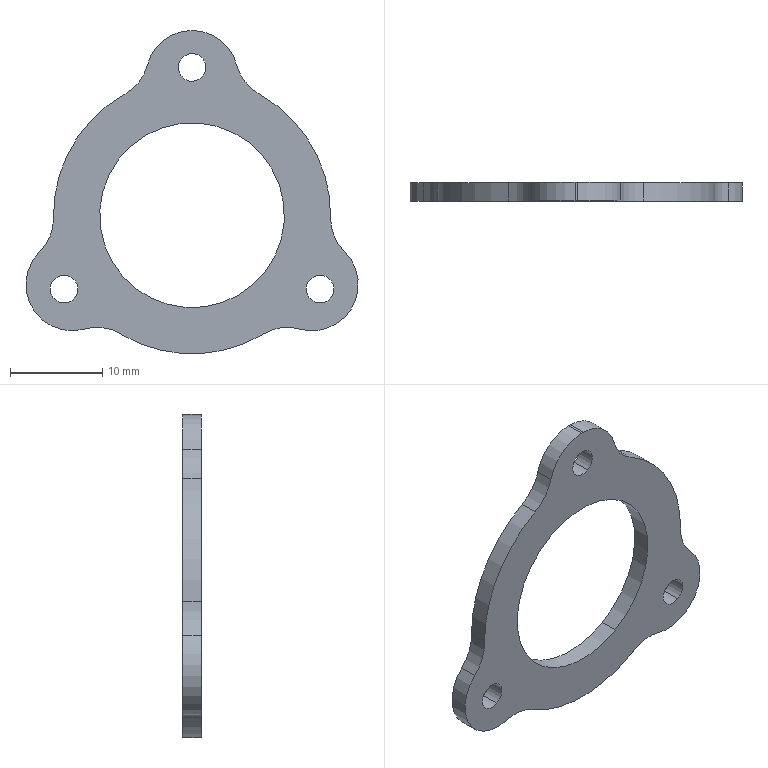Component | SolidWorks | NozzleGasket1-1 | 1 solid | 27 faces | box 35.98 x 2 x 35 mm | volume 1008 mm3 | cylinder 25 | plane 2 | commonest cylinder face diameters 10 x12 3 x6 30 x4 20 x2 40 x1
build123d program:
from build123d import *

# Parameters (mm, degrees)
SKETCH1_R           = 10
BOSS_EXTRUDE1_DEPTH = 2
FILLET1_R           = 5
CUT_EXTRUDE1_REACH  = 28.976
SKETCH2_R           = 1.5


with BuildPart() as part:
    # Sketch1 → Boss-Extrude1 (new body)
    with BuildSketch(Plane.XY):
        with BuildLine():
            ThreePointArc((4.93, 14.167), (0, 20), (-4.93, 14.167))
            ThreePointArc((-4.93, 14.167), (-12.991, 7.499), (-14.733, -2.815))
            ThreePointArc((-14.733, -2.815), (-17.319, -10.001), (-9.802, -11.354))
            ThreePointArc((-9.802, -11.354), (0.001646, -15), (9.805, -11.352))
            ThreePointArc((9.805, -11.352), (17.322, -9.999), (14.734, -2.812))
            ThreePointArc((14.734, -2.812), (12.99, 7.501), (4.93, 14.167))
        make_face()
        Circle(SKETCH1_R, mode=Mode.SUBTRACT)
    extrude(amount=BOSS_EXTRUDE1_DEPTH)

    # Fillet1
    fillet1_edges = [part.edges().sort_by_distance(p)[0] for p in [
        (14.734, -2.812, 1),
        (9.805, -11.352, 1),
        (-9.802, -11.354, 1),
        (-14.733, -2.815, 1),
        (-4.93, 14.167, 1),
        (4.93, 14.167, 1),
    ]]
    fillet(fillet1_edges, radius=FILLET1_R)

    # Sketch2 → Cut-Extrude1 (cut, up to next)
    with BuildSketch(Plane.XY.offset(2), mode=Mode.PRIVATE) as cut_extrude1_sk1:
        with Locations((0, 16)):
            Circle(SKETCH2_R)
    cut_extrude1_tool1 = extrude(cut_extrude1_sk1.sketch, amount=-CUT_EXTRUDE1_REACH, mode=Mode.PRIVATE) & part.part
    # Sketch2 → Cut-Extrude1 (cut, up to next)
    with BuildSketch(Plane.XY.offset(2), mode=Mode.PRIVATE) as cut_extrude1_sk2:
        with Locations((13.856, -8)):
            Circle(SKETCH2_R)
    cut_extrude1_tool2 = extrude(cut_extrude1_sk2.sketch, amount=-CUT_EXTRUDE1_REACH, mode=Mode.PRIVATE) & part.part
    # Sketch2 → Cut-Extrude1 (cut, up to next)
    with BuildSketch(Plane.XY.offset(2), mode=Mode.PRIVATE) as cut_extrude1_sk3:
        with Locations((-13.856, -8)):
            Circle(SKETCH2_R)
    cut_extrude1_tool3 = extrude(cut_extrude1_sk3.sketch, amount=-CUT_EXTRUDE1_REACH, mode=Mode.PRIVATE) & part.part
    add(cut_extrude1_tool1.solids().sort_by_distance((0, 16, 2))[0], mode=Mode.SUBTRACT)
    add(cut_extrude1_tool2.solids().sort_by_distance((13.856, -8, 2))[0], mode=Mode.SUBTRACT)
    add(cut_extrude1_tool3.solids().sort_by_distance((-13.856, -8, 2))[0], mode=Mode.SUBTRACT)


solid = part.part

# Placed as in the assembly
solid = solid.moved(Location((-5.982, -9.494, 160.001), (90, 0, 0)))
STEP:
#1=COLOUR_RGB('',0.7922,0.8196,0.9333);
#2=FILL_AREA_STYLE_COLOUR('',#1);
#3=FILL_AREA_STYLE('',(#2));
#4=SURFACE_STYLE_FILL_AREA(#3);
#5=SURFACE_SIDE_STYLE('',(#4));
#6=SURFACE_STYLE_USAGE(.BOTH.,#5);
#7=PRESENTATION_STYLE_ASSIGNMENT((#6));
#8=CARTESIAN_POINT('',(-0.8105,-0.3738,6.035));
#9=VERTEX_POINT('',#8);
#10=CARTESIAN_POINT('',(-0.7515,-0.3738,5.933));
#11=VERTEX_POINT('',#10);
#12=CARTESIAN_POINT('',(-0.781,-0.3738,5.984));
#13=DIRECTION('',(0.,1.,0.));
#14=DIRECTION('',(-0.5,0.,0.866));
#15=AXIS2_PLACEMENT_3D('',#12,#13,#14);
#16=CIRCLE('',#15,0.05906);
#17=EDGE_CURVE('',#9,#11,#16,.T.);
#18=ORIENTED_EDGE('',*,*,#17,.T.);
#19=CARTESIAN_POINT('',(-0.7515,-0.4525,5.933));
#20=VERTEX_POINT('',#19);
#21=CARTESIAN_POINT('',(-0.7515,-0.3737,5.933));
#22=DIRECTION('',(-0.,-1.,-0.));
#23=VECTOR('',#22,39.37);
#24=LINE('',#21,#23);
#25=EDGE_CURVE('',#11,#20,#24,.T.);
#26=ORIENTED_EDGE('',*,*,#25,.T.);
#27=CARTESIAN_POINT('',(-0.8105,-0.4525,6.035));
#28=VERTEX_POINT('',#27);
#29=CARTESIAN_POINT('',(-0.781,-0.4525,5.984));
#30=DIRECTION('',(-0.,-1.,-0.));
#31=DIRECTION('',(-0.5,0.,0.866));
#32=AXIS2_PLACEMENT_3D('',#29,#30,#31);
#33=CIRCLE('',#32,0.05906);
#34=EDGE_CURVE('',#20,#28,#33,.T.);
#35=ORIENTED_EDGE('',*,*,#34,.T.);
#36=CARTESIAN_POINT('',(-0.8105,-0.3737,6.035));
#37=DIRECTION('',(-0.,-1.,-0.));
#38=VECTOR('',#37,39.37);
#39=LINE('',#36,#38);
#40=EDGE_CURVE('',#9,#28,#39,.T.);
#41=ORIENTED_EDGE('',*,*,#40,.F.);
#42=EDGE_LOOP('',(#18,#26,#35,#41));
#43=FACE_OUTER_BOUND('',#42,.T.);
#44=CARTESIAN_POINT('',(-0.781,-0.3737,5.984));
#45=DIRECTION('',(-0.,-1.,-0.));
#46=DIRECTION('',(-0.5,0.,0.866));
#47=AXIS2_PLACEMENT_3D('',#44,#45,#46);
#48=CYLINDRICAL_SURFACE('',#47,0.05906);
#49=ADVANCED_FACE('',(#43),#48,.F.);
#50=CARTESIAN_POINT('',(-0.265,-0.3738,6.98));
#51=VERTEX_POINT('',#50);
#52=CARTESIAN_POINT('',(-0.2059,-0.3738,6.878));
#53=VERTEX_POINT('',#52);
#54=CARTESIAN_POINT('',(-0.2355,-0.3738,6.929));
#55=DIRECTION('',(0.,1.,0.));
#56=DIRECTION('',(-0.5,0.,0.866));
#57=AXIS2_PLACEMENT_3D('',#54,#55,#56);
#58=CIRCLE('',#57,0.05906);
#59=EDGE_CURVE('',#51,#53,#58,.T.);
#60=ORIENTED_EDGE('',*,*,#59,.T.);
#61=CARTESIAN_POINT('',(-0.2059,-0.4525,6.878));
#62=VERTEX_POINT('',#61);
#63=CARTESIAN_POINT('',(-0.2059,-0.3737,6.878));
#64=DIRECTION('',(-0.,-1.,-0.));
#65=VECTOR('',#64,39.37);
#66=LINE('',#63,#65);
#67=EDGE_CURVE('',#53,#62,#66,.T.);
#68=ORIENTED_EDGE('',*,*,#67,.T.);
#69=CARTESIAN_POINT('',(-0.265,-0.4525,6.98));
#70=VERTEX_POINT('',#69);
#71=CARTESIAN_POINT('',(-0.2355,-0.4525,6.929));
#72=DIRECTION('',(-0.,-1.,-0.));
#73=DIRECTION('',(-0.5,0.,0.866));
#74=AXIS2_PLACEMENT_3D('',#71,#72,#73);
#75=CIRCLE('',#74,0.05906);
#76=EDGE_CURVE('',#62,#70,#75,.T.);
#77=ORIENTED_EDGE('',*,*,#76,.T.);
#78=CARTESIAN_POINT('',(-0.265,-0.3737,6.98));
#79=DIRECTION('',(-0.,-1.,-0.));
#80=VECTOR('',#79,39.37);
#81=LINE('',#78,#80);
#82=EDGE_CURVE('',#51,#70,#81,.T.);
#83=ORIENTED_EDGE('',*,*,#82,.F.);
#84=EDGE_LOOP('',(#60,#68,#77,#83));
#85=FACE_OUTER_BOUND('',#84,.T.);
#86=CARTESIAN_POINT('',(-0.2355,-0.3737,6.929));
#87=DIRECTION('',(-0.,-1.,-0.));
#88=DIRECTION('',(-0.5,0.,0.866));
#89=AXIS2_PLACEMENT_3D('',#86,#87,#88);
#90=CYLINDRICAL_SURFACE('',#89,0.05906);
#91=ADVANCED_FACE('',(#85),#90,.F.);
#92=CARTESIAN_POINT('',(0.2805,-0.3738,6.035));
#93=VERTEX_POINT('',#92);
#94=CARTESIAN_POINT('',(0.3396,-0.3738,5.933));
#95=VERTEX_POINT('',#94);
#96=CARTESIAN_POINT('',(0.3101,-0.3738,5.984));
#97=DIRECTION('',(0.,1.,0.));
#98=DIRECTION('',(-0.5,0.,0.866));
#99=AXIS2_PLACEMENT_3D('',#96,#97,#98);
#100=CIRCLE('',#99,0.05906);
#101=EDGE_CURVE('',#93,#95,#100,.T.);
#102=ORIENTED_EDGE('',*,*,#101,.T.);
#103=CARTESIAN_POINT('',(0.3396,-0.4525,5.933));
#104=VERTEX_POINT('',#103);
#105=CARTESIAN_POINT('',(0.3396,-0.3737,5.933));
#106=DIRECTION('',(-0.,-1.,-0.));
#107=VECTOR('',#106,39.37);
#108=LINE('',#105,#107);
#109=EDGE_CURVE('',#95,#104,#108,.T.);
#110=ORIENTED_EDGE('',*,*,#109,.T.);
#111=CARTESIAN_POINT('',(0.2805,-0.4525,6.035));
#112=VERTEX_POINT('',#111);
#113=CARTESIAN_POINT('',(0.3101,-0.4525,5.984));
#114=DIRECTION('',(-0.,-1.,-0.));
#115=DIRECTION('',(-0.5,0.,0.866));
#116=AXIS2_PLACEMENT_3D('',#113,#114,#115);
#117=CIRCLE('',#116,0.05906);
#118=EDGE_CURVE('',#104,#112,#117,.T.);
#119=ORIENTED_EDGE('',*,*,#118,.T.);
#120=CARTESIAN_POINT('',(0.2805,-0.3737,6.035));
#121=DIRECTION('',(-0.,-1.,-0.));
#122=VECTOR('',#121,39.37);
#123=LINE('',#120,#122);
#124=EDGE_CURVE('',#93,#112,#123,.T.);
#125=ORIENTED_EDGE('',*,*,#124,.F.);
#126=EDGE_LOOP('',(#102,#110,#119,#125));
#127=FACE_OUTER_BOUND('',#126,.T.);
#128=CARTESIAN_POINT('',(0.3101,-0.3737,5.984));
#129=DIRECTION('',(-0.,-1.,-0.));
#130=DIRECTION('',(-0.5,0.,0.866));
#131=AXIS2_PLACEMENT_3D('',#128,#129,#130);
#132=CYLINDRICAL_SURFACE('',#131,0.05906);
#133=ADVANCED_FACE('',(#127),#132,.F.);
#134=CARTESIAN_POINT('',(0.07226,-0.3738,5.795));
#135=VERTEX_POINT('',#134);
#136=CARTESIAN_POINT('',(0.06914,-0.3738,5.793));
#137=VERTEX_POINT('',#136);
#138=CARTESIAN_POINT('',(0.1707,-0.3738,5.625));
#139=DIRECTION('',(-0.,-1.,-0.));
#140=DIRECTION('',(-0.5,-0.,0.866));
#141=AXIS2_PLACEMENT_3D('',#138,#139,#140);
#142=CIRCLE('',#141,0.1969);
#143=EDGE_CURVE('',#135,#137,#142,.T.);
#144=ORIENTED_EDGE('',*,*,#143,.F.);
#145=CARTESIAN_POINT('',(0.07226,-0.4525,5.795));
#146=VERTEX_POINT('',#145);
#147=CARTESIAN_POINT('',(0.07226,-0.4525,5.795));
#148=DIRECTION('',(-0.,-1.,-0.));
#149=VECTOR('',#148,39.37);
#150=LINE('',#147,#149);
#151=EDGE_CURVE('',#135,#146,#150,.T.);
#152=ORIENTED_EDGE('',*,*,#151,.T.);
#153=CARTESIAN_POINT('',(0.06914,-0.4525,5.793));
#154=VERTEX_POINT('',#153);
#155=CARTESIAN_POINT('',(0.1707,-0.4525,5.625));
#156=DIRECTION('',(0.,1.,0.));
#157=DIRECTION('',(-0.5,-0.,0.866));
#158=AXIS2_PLACEMENT_3D('',#155,#156,#157);
#159=CIRCLE('',#158,0.1969);
#160=EDGE_CURVE('',#154,#146,#159,.T.);
#161=ORIENTED_EDGE('',*,*,#160,.F.);
#162=CARTESIAN_POINT('',(0.06914,-0.4525,5.793));
#163=DIRECTION('',(-0.,-1.,-0.));
#164=VECTOR('',#163,39.37);
#165=LINE('',#162,#164);
#166=EDGE_CURVE('',#137,#154,#165,.T.);
#167=ORIENTED_EDGE('',*,*,#166,.F.);
#168=EDGE_LOOP('',(#144,#152,#161,#167));
#169=FACE_OUTER_BOUND('',#168,.T.);
#170=CARTESIAN_POINT('',(0.1707,-0.4525,5.625));
#171=DIRECTION('',(-0.,-1.,-0.));
#172=DIRECTION('',(-0.5,-0.,0.866));
#173=AXIS2_PLACEMENT_3D('',#170,#171,#172);
#174=CYLINDRICAL_SURFACE('',#173,0.1969);
#175=ADVANCED_FACE('',(#169),#174,.F.);
#176=CARTESIAN_POINT('',(-0.03862,-0.4525,5.958));
#177=VERTEX_POINT('',#176);
#178=CARTESIAN_POINT('',(-0.4323,-0.4525,6.64));
#179=VERTEX_POINT('',#178);
#180=CARTESIAN_POINT('',(-0.2355,-0.4525,6.299));
#181=DIRECTION('',(-0.,-1.,-0.));
#182=DIRECTION('',(-0.5,-0.,0.866));
#183=AXIS2_PLACEMENT_3D('',#180,#181,#182);
#184=CIRCLE('',#183,0.3937);
#185=EDGE_CURVE('',#177,#179,#184,.T.);
#186=ORIENTED_EDGE('',*,*,#185,.T.);
#187=CARTESIAN_POINT('',(-0.4323,-0.3738,6.64));
#188=VERTEX_POINT('',#187);
#189=CARTESIAN_POINT('',(-0.4323,-0.4525,6.64));
#190=DIRECTION('',(0.,1.,0.));
#191=VECTOR('',#190,39.37);
#192=LINE('',#189,#191);
#193=EDGE_CURVE('',#179,#188,#192,.T.);
#194=ORIENTED_EDGE('',*,*,#193,.T.);
#195=CARTESIAN_POINT('',(-0.03862,-0.3738,5.958));
#196=VERTEX_POINT('',#195);
#197=CARTESIAN_POINT('',(-0.2355,-0.3738,6.299));
#198=DIRECTION('',(-0.,-1.,-0.));
#199=DIRECTION('',(-0.5,-0.,0.866));
#200=AXIS2_PLACEMENT_3D('',#197,#198,#199);
#201=CIRCLE('',#200,0.3937);
#202=EDGE_CURVE('',#196,#188,#201,.T.);
#203=ORIENTED_EDGE('',*,*,#202,.F.);
#204=CARTESIAN_POINT('',(-0.03862,-0.4525,5.958));
#205=DIRECTION('',(0.,1.,0.));
#206=VECTOR('',#205,39.37);
#207=LINE('',#204,#206);
#208=EDGE_CURVE('',#177,#196,#207,.T.);
#209=ORIENTED_EDGE('',*,*,#208,.F.);
#210=EDGE_LOOP('',(#186,#194,#203,#209));
#211=FACE_OUTER_BOUND('',#210,.T.);
#212=CARTESIAN_POINT('',(-0.2355,-0.4525,6.299));
#213=DIRECTION('',(0.,1.,0.));
#214=DIRECTION('',(0.5,0.,-0.866));
#215=AXIS2_PLACEMENT_3D('',#212,#213,#214);
#216=CYLINDRICAL_SURFACE('',#215,0.3937);
#217=ADVANCED_FACE('',(#211),#216,.F.);
#218=CARTESIAN_POINT('',(0.3744,-0.4525,5.834));
#219=VERTEX_POINT('',#218);
#220=CARTESIAN_POINT('',(0.4139,-0.4525,6.144));
#221=VERTEX_POINT('',#220);
#222=CARTESIAN_POINT('',(0.276,-0.4525,6.004));
#223=DIRECTION('',(-0.,-1.,-0.));
#224=DIRECTION('',(-0.5,-0.,0.866));
#225=AXIS2_PLACEMENT_3D('',#222,#223,#224);
#226=CIRCLE('',#225,0.1969);
#227=EDGE_CURVE('',#219,#221,#226,.T.);
#228=ORIENTED_EDGE('',*,*,#227,.F.);
#229=CARTESIAN_POINT('',(0.3744,-0.3738,5.834));
#230=VERTEX_POINT('',#229);
#231=CARTESIAN_POINT('',(0.3744,-0.4525,5.834));
#232=DIRECTION('',(0.,1.,0.));
#233=VECTOR('',#232,39.37);
#234=LINE('',#231,#233);
#235=EDGE_CURVE('',#219,#230,#234,.T.);
#236=ORIENTED_EDGE('',*,*,#235,.T.);
#237=CARTESIAN_POINT('',(0.4139,-0.3738,6.144));
#238=VERTEX_POINT('',#237);
#239=CARTESIAN_POINT('',(0.276,-0.3738,6.004));
#240=DIRECTION('',(-0.,-1.,-0.));
#241=DIRECTION('',(-0.5,-0.,0.866));
#242=AXIS2_PLACEMENT_3D('',#239,#240,#241);
#243=CIRCLE('',#242,0.1969);
#244=EDGE_CURVE('',#230,#238,#243,.T.);
#245=ORIENTED_EDGE('',*,*,#244,.T.);
#246=CARTESIAN_POINT('',(0.4139,-0.4525,6.144));
#247=DIRECTION('',(-0.,-1.,-0.));
#248=VECTOR('',#247,39.37);
#249=LINE('',#246,#248);
#250=EDGE_CURVE('',#238,#221,#249,.T.);
#251=ORIENTED_EDGE('',*,*,#250,.T.);
#252=EDGE_LOOP('',(#228,#236,#245,#251));
#253=FACE_OUTER_BOUND('',#252,.T.);
#254=CARTESIAN_POINT('',(0.276,-0.4525,6.004));
#255=DIRECTION('',(0.,1.,0.));
#256=DIRECTION('',(0.5,0.,-0.866));
#257=AXIS2_PLACEMENT_3D('',#254,#255,#256);
#258=CYLINDRICAL_SURFACE('',#257,0.1969);
#259=ADVANCED_FACE('',(#253),#258,.T.);
#260=CARTESIAN_POINT('',(0.05981,-0.4525,5.788));
#261=VERTEX_POINT('',#260);
#262=CARTESIAN_POINT('',(-0.2355,-0.4525,6.299));
#263=DIRECTION('',(-0.,-1.,-0.));
#264=DIRECTION('',(-0.5,-0.,0.866));
#265=AXIS2_PLACEMENT_3D('',#262,#263,#264);
#266=CIRCLE('',#265,0.5906);
#267=EDGE_CURVE('',#261,#154,#266,.T.);
#268=ORIENTED_EDGE('',*,*,#267,.F.);
#269=CARTESIAN_POINT('',(0.05981,-0.3738,5.788));
#270=VERTEX_POINT('',#269);
#271=CARTESIAN_POINT('',(0.05981,-0.4525,5.788));
#272=DIRECTION('',(0.,1.,0.));
#273=VECTOR('',#272,39.37);
#274=LINE('',#271,#273);
#275=EDGE_CURVE('',#261,#270,#274,.T.);
#276=ORIENTED_EDGE('',*,*,#275,.T.);
#277=CARTESIAN_POINT('',(-0.2355,-0.3738,6.299));
#278=DIRECTION('',(-0.,-1.,-0.));
#279=DIRECTION('',(-0.5,-0.,0.866));
#280=AXIS2_PLACEMENT_3D('',#277,#278,#279);
#281=CIRCLE('',#280,0.5906);
#282=EDGE_CURVE('',#270,#137,#281,.T.);
#283=ORIENTED_EDGE('',*,*,#282,.T.);
#284=ORIENTED_EDGE('',*,*,#166,.T.);
#285=EDGE_LOOP('',(#268,#276,#283,#284));
#286=FACE_OUTER_BOUND('',#285,.T.);
#287=CARTESIAN_POINT('',(-0.2355,-0.4525,6.299));
#288=DIRECTION('',(0.,1.,0.));
#289=DIRECTION('',(0.5,0.,-0.866));
#290=AXIS2_PLACEMENT_3D('',#287,#288,#289);
#291=CYLINDRICAL_SURFACE('',#290,0.5906);
#292=ADVANCED_FACE('',(#286),#291,.T.);
#293=CARTESIAN_POINT('',(-0.5214,-0.4525,6.816));
#294=VERTEX_POINT('',#293);
#295=CARTESIAN_POINT('',(-0.8259,-0.4525,6.288));
#296=VERTEX_POINT('',#295);
#297=CARTESIAN_POINT('',(-0.2355,-0.4525,6.299));
#298=DIRECTION('',(-0.,-1.,-0.));
#299=DIRECTION('',(-0.5,-0.,0.866));
#300=AXIS2_PLACEMENT_3D('',#297,#298,#299);
#301=CIRCLE('',#300,0.5906);
#302=EDGE_CURVE('',#294,#296,#301,.T.);
#303=ORIENTED_EDGE('',*,*,#302,.F.);
#304=CARTESIAN_POINT('',(-0.5214,-0.3738,6.816));
#305=VERTEX_POINT('',#304);
#306=CARTESIAN_POINT('',(-0.5214,-0.4525,6.816));
#307=DIRECTION('',(0.,1.,0.));
#308=VECTOR('',#307,39.37);
#309=LINE('',#306,#308);
#310=EDGE_CURVE('',#294,#305,#309,.T.);
#311=ORIENTED_EDGE('',*,*,#310,.T.);
#312=CARTESIAN_POINT('',(-0.8259,-0.3738,6.288));
#313=VERTEX_POINT('',#312);
#314=CARTESIAN_POINT('',(-0.2355,-0.3738,6.299));
#315=DIRECTION('',(-0.,-1.,-0.));
#316=DIRECTION('',(-0.5,-0.,0.866));
#317=AXIS2_PLACEMENT_3D('',#314,#315,#316);
#318=CIRCLE('',#317,0.5906);
#319=EDGE_CURVE('',#305,#313,#318,.T.);
#320=ORIENTED_EDGE('',*,*,#319,.T.);
#321=CARTESIAN_POINT('',(-0.8259,-0.4525,6.288));
#322=DIRECTION('',(-0.,-1.,-0.));
#323=VECTOR('',#322,39.37);
#324=LINE('',#321,#323);
#325=EDGE_CURVE('',#313,#296,#324,.T.);
#326=ORIENTED_EDGE('',*,*,#325,.T.);
#327=EDGE_LOOP('',(#303,#311,#320,#326));
#328=FACE_OUTER_BOUND('',#327,.T.);
#329=CARTESIAN_POINT('',(-0.2355,-0.4525,6.299));
#330=DIRECTION('',(0.,1.,0.));
#331=DIRECTION('',(0.5,0.,-0.866));
#332=AXIS2_PLACEMENT_3D('',#329,#330,#331);
#333=CYLINDRICAL_SURFACE('',#332,0.5906);
#334=ADVANCED_FACE('',(#328),#333,.T.);
#335=CARTESIAN_POINT('',(-0.8848,-0.3738,6.144));
#336=VERTEX_POINT('',#335);
#337=CARTESIAN_POINT('',(-0.6942,-0.3738,5.814));
#338=VERTEX_POINT('',#337);
#339=CARTESIAN_POINT('',(-0.7469,-0.3738,6.004));
#340=DIRECTION('',(-0.,-1.,-0.));
#341=DIRECTION('',(-0.5,-0.,0.866));
#342=AXIS2_PLACEMENT_3D('',#339,#340,#341);
#343=CIRCLE('',#342,0.1969);
#344=EDGE_CURVE('',#336,#338,#343,.T.);
#345=ORIENTED_EDGE('',*,*,#344,.T.);
#346=CARTESIAN_POINT('',(-0.6942,-0.4525,5.814));
#347=VERTEX_POINT('',#346);
#348=CARTESIAN_POINT('',(-0.6942,-0.4525,5.814));
#349=DIRECTION('',(-0.,-1.,-0.));
#350=VECTOR('',#349,39.37);
#351=LINE('',#348,#350);
#352=EDGE_CURVE('',#338,#347,#351,.T.);
#353=ORIENTED_EDGE('',*,*,#352,.T.);
#354=CARTESIAN_POINT('',(-0.8848,-0.4525,6.144));
#355=VERTEX_POINT('',#354);
#356=CARTESIAN_POINT('',(-0.7469,-0.4525,6.004));
#357=DIRECTION('',(-0.,-1.,-0.));
#358=DIRECTION('',(-0.5,-0.,0.866));
#359=AXIS2_PLACEMENT_3D('',#356,#357,#358);
#360=CIRCLE('',#359,0.1969);
#361=EDGE_CURVE('',#355,#347,#360,.T.);
#362=ORIENTED_EDGE('',*,*,#361,.F.);
#363=CARTESIAN_POINT('',(-0.8848,-0.4525,6.144));
#364=DIRECTION('',(0.,1.,0.));
#365=VECTOR('',#364,39.37);
#366=LINE('',#363,#365);
#367=EDGE_CURVE('',#355,#336,#366,.T.);
#368=ORIENTED_EDGE('',*,*,#367,.T.);
#369=EDGE_LOOP('',(#345,#353,#362,#368));
#370=FACE_OUTER_BOUND('',#369,.T.);
#371=CARTESIAN_POINT('',(-0.7469,-0.4525,6.004));
#372=DIRECTION('',(0.,1.,0.));
#373=DIRECTION('',(0.5,0.,-0.866));
#374=AXIS2_PLACEMENT_3D('',#371,#372,#373);
#375=CYLINDRICAL_SURFACE('',#374,0.1969);
#376=ADVANCED_FACE('',(#370),#375,.T.);
#377=ORIENTED_EDGE('',*,*,#275,.F.);
#378=CARTESIAN_POINT('',(-0.54,-0.4525,5.793));
#379=VERTEX_POINT('',#378);
#380=CARTESIAN_POINT('',(-0.2355,-0.4525,6.299));
#381=DIRECTION('',(-0.,-1.,-0.));
#382=DIRECTION('',(-0.5,-0.,0.866));
#383=AXIS2_PLACEMENT_3D('',#380,#381,#382);
#384=CIRCLE('',#383,0.5906);
#385=EDGE_CURVE('',#379,#261,#384,.T.);
#386=ORIENTED_EDGE('',*,*,#385,.F.);
#387=CARTESIAN_POINT('',(-0.54,-0.3738,5.793));
#388=VERTEX_POINT('',#387);
#389=CARTESIAN_POINT('',(-0.54,-0.4525,5.793));
#390=DIRECTION('',(0.,1.,0.));
#391=VECTOR('',#390,39.37);
#392=LINE('',#389,#391);
#393=EDGE_CURVE('',#379,#388,#392,.T.);
#394=ORIENTED_EDGE('',*,*,#393,.T.);
#395=CARTESIAN_POINT('',(-0.2355,-0.3738,6.299));
#396=DIRECTION('',(-0.,-1.,-0.));
#397=DIRECTION('',(-0.5,-0.,0.866));
#398=AXIS2_PLACEMENT_3D('',#395,#396,#397);
#399=CIRCLE('',#398,0.5906);
#400=EDGE_CURVE('',#388,#270,#399,.T.);
#401=ORIENTED_EDGE('',*,*,#400,.T.);
#402=EDGE_LOOP('',(#377,#386,#394,#401));
#403=FACE_OUTER_BOUND('',#402,.T.);
#404=CARTESIAN_POINT('',(-0.2355,-0.4525,6.299));
#405=DIRECTION('',(0.,1.,0.));
#406=DIRECTION('',(0.5,0.,-0.866));
#407=AXIS2_PLACEMENT_3D('',#404,#405,#406);
#408=CYLINDRICAL_SURFACE('',#407,0.5906);
#409=ADVANCED_FACE('',(#403),#408,.T.);
#410=ORIENTED_EDGE('',*,*,#235,.F.);
#411=CARTESIAN_POINT('',(0.2233,-0.4525,5.814));
#412=VERTEX_POINT('',#411);
#413=CARTESIAN_POINT('',(0.276,-0.4525,6.004));
#414=DIRECTION('',(-0.,-1.,-0.));
#415=DIRECTION('',(-0.5,-0.,0.866));
#416=AXIS2_PLACEMENT_3D('',#413,#414,#415);
#417=CIRCLE('',#416,0.1969);
#418=EDGE_CURVE('',#412,#219,#417,.T.);
#419=ORIENTED_EDGE('',*,*,#418,.F.);
#420=CARTESIAN_POINT('',(0.2233,-0.3738,5.814));
#421=VERTEX_POINT('',#420);
#422=CARTESIAN_POINT('',(0.2233,-0.4525,5.814));
#423=DIRECTION('',(0.,1.,0.));
#424=VECTOR('',#423,39.37);
#425=LINE('',#422,#424);
#426=EDGE_CURVE('',#412,#421,#425,.T.);
#427=ORIENTED_EDGE('',*,*,#426,.T.);
#428=CARTESIAN_POINT('',(0.276,-0.3738,6.004));
#429=DIRECTION('',(-0.,-1.,-0.));
#430=DIRECTION('',(-0.5,-0.,0.866));
#431=AXIS2_PLACEMENT_3D('',#428,#429,#430);
#432=CIRCLE('',#431,0.1969);
#433=EDGE_CURVE('',#421,#230,#432,.T.);
#434=ORIENTED_EDGE('',*,*,#433,.T.);
#435=EDGE_LOOP('',(#410,#419,#427,#434));
#436=FACE_OUTER_BOUND('',#435,.T.);
#437=CARTESIAN_POINT('',(0.276,-0.4525,6.004));
#438=DIRECTION('',(0.,1.,0.));
#439=DIRECTION('',(0.5,0.,-0.866));
#440=AXIS2_PLACEMENT_3D('',#437,#438,#439);
#441=CYLINDRICAL_SURFACE('',#440,0.1969);
#442=ADVANCED_FACE('',(#436),#441,.T.);
#443=CARTESIAN_POINT('',(0.355,-0.3738,6.288));
#444=VERTEX_POINT('',#443);
#445=CARTESIAN_POINT('',(0.05039,-0.3738,6.816));
#446=VERTEX_POINT('',#445);
#447=CARTESIAN_POINT('',(-0.2355,-0.3738,6.299));
#448=DIRECTION('',(-0.,-1.,-0.));
#449=DIRECTION('',(-0.5,-0.,0.866));
#450=AXIS2_PLACEMENT_3D('',#447,#448,#449);
#451=CIRCLE('',#450,0.5906);
#452=EDGE_CURVE('',#444,#446,#451,.T.);
#453=ORIENTED_EDGE('',*,*,#452,.T.);
#454=CARTESIAN_POINT('',(0.05039,-0.4525,6.816));
#455=VERTEX_POINT('',#454);
#456=CARTESIAN_POINT('',(0.05039,-0.4525,6.816));
#457=DIRECTION('',(-0.,-1.,-0.));
#458=VECTOR('',#457,39.37);
#459=LINE('',#456,#458);
#460=EDGE_CURVE('',#446,#455,#459,.T.);
#461=ORIENTED_EDGE('',*,*,#460,.T.);
#462=CARTESIAN_POINT('',(0.355,-0.4525,6.288));
#463=VERTEX_POINT('',#462);
#464=CARTESIAN_POINT('',(-0.2355,-0.4525,6.299));
#465=DIRECTION('',(-0.,-1.,-0.));
#466=DIRECTION('',(-0.5,-0.,0.866));
#467=AXIS2_PLACEMENT_3D('',#464,#465,#466);
#468=CIRCLE('',#467,0.5906);
#469=EDGE_CURVE('',#463,#455,#468,.T.);
#470=ORIENTED_EDGE('',*,*,#469,.F.);
#471=CARTESIAN_POINT('',(0.355,-0.4525,6.288));
#472=DIRECTION('',(0.,1.,0.));
#473=VECTOR('',#472,39.37);
#474=LINE('',#471,#473);
#475=EDGE_CURVE('',#463,#444,#474,.T.);
#476=ORIENTED_EDGE('',*,*,#475,.T.);
#477=EDGE_LOOP('',(#453,#461,#470,#476));
#478=FACE_OUTER_BOUND('',#477,.T.);
#479=CARTESIAN_POINT('',(-0.2355,-0.4525,6.299));
#480=DIRECTION('',(0.,1.,0.));
#481=DIRECTION('',(0.5,0.,-0.866));
#482=AXIS2_PLACEMENT_3D('',#479,#480,#481);
#483=CYLINDRICAL_SURFACE('',#482,0.5906);
#484=ADVANCED_FACE('',(#478),#483,.T.);
#485=CARTESIAN_POINT('',(-0.04493,-0.4525,6.939));
#486=VERTEX_POINT('',#485);
#487=CARTESIAN_POINT('',(-0.2313,-0.4525,7.087));
#488=VERTEX_POINT('',#487);
#489=CARTESIAN_POINT('',(-0.2355,-0.4525,6.89));
#490=DIRECTION('',(-0.,-1.,-0.));
#491=DIRECTION('',(-0.5,-0.,0.866));
#492=AXIS2_PLACEMENT_3D('',#489,#490,#491);
#493=CIRCLE('',#492,0.1969);
#494=EDGE_CURVE('',#486,#488,#493,.T.);
#495=ORIENTED_EDGE('',*,*,#494,.F.);
#496=CARTESIAN_POINT('',(-0.04493,-0.3738,6.939));
#497=VERTEX_POINT('',#496);
#498=CARTESIAN_POINT('',(-0.04493,-0.4525,6.939));
#499=DIRECTION('',(0.,1.,0.));
#500=VECTOR('',#499,39.37);
#501=LINE('',#498,#500);
#502=EDGE_CURVE('',#486,#497,#501,.T.);
#503=ORIENTED_EDGE('',*,*,#502,.T.);
#504=CARTESIAN_POINT('',(-0.2313,-0.3738,7.087));
#505=VERTEX_POINT('',#504);
#506=CARTESIAN_POINT('',(-0.2355,-0.3738,6.89));
#507=DIRECTION('',(-0.,-1.,-0.));
#508=DIRECTION('',(-0.5,-0.,0.866));
#509=AXIS2_PLACEMENT_3D('',#506,#507,#508);
#510=CIRCLE('',#509,0.1969);
#511=EDGE_CURVE('',#497,#505,#510,.T.);
#512=ORIENTED_EDGE('',*,*,#511,.T.);
#513=CARTESIAN_POINT('',(-0.2313,-0.4525,7.087));
#514=DIRECTION('',(0.,1.,0.));
#515=VECTOR('',#514,39.37);
#516=LINE('',#513,#515);
#517=EDGE_CURVE('',#488,#505,#516,.T.);
#518=ORIENTED_EDGE('',*,*,#517,.F.);
#519=EDGE_LOOP('',(#495,#503,#512,#518));
#520=FACE_OUTER_BOUND('',#519,.T.);
#521=CARTESIAN_POINT('',(-0.2355,-0.4525,6.89));
#522=DIRECTION('',(0.,1.,0.));
#523=DIRECTION('',(0.5,0.,-0.866));
#524=AXIS2_PLACEMENT_3D('',#521,#522,#523);
#525=CYLINDRICAL_SURFACE('',#524,0.1969);
#526=ADVANCED_FACE('',(#520),#525,.T.);
#527=CARTESIAN_POINT('',(-0.2398,-0.3738,7.087));
#528=VERTEX_POINT('',#527);
#529=CARTESIAN_POINT('',(-0.2355,-0.3738,6.299));
#530=DIRECTION('',(-0.,-1.,-0.));
#531=DIRECTION('',(-0.5,-0.,0.866));
#532=AXIS2_PLACEMENT_3D('',#529,#530,#531);
#533=CIRCLE('',#532,0.7874);
#534=EDGE_CURVE('',#505,#528,#533,.T.);
#535=ORIENTED_EDGE('',*,*,#534,.T.);
#536=CARTESIAN_POINT('',(-0.2398,-0.4525,7.087));
#537=VERTEX_POINT('',#536);
#538=CARTESIAN_POINT('',(-0.2398,-0.4525,7.087));
#539=DIRECTION('',(0.,1.,0.));
#540=VECTOR('',#539,39.37);
#541=LINE('',#538,#540);
#542=EDGE_CURVE('',#537,#528,#541,.T.);
#543=ORIENTED_EDGE('',*,*,#542,.F.);
#544=CARTESIAN_POINT('',(-0.2355,-0.4525,6.299));
#545=DIRECTION('',(-0.,-1.,-0.));
#546=DIRECTION('',(-0.5,-0.,0.866));
#547=AXIS2_PLACEMENT_3D('',#544,#545,#546);
#548=CIRCLE('',#547,0.7874);
#549=EDGE_CURVE('',#488,#537,#548,.T.);
#550=ORIENTED_EDGE('',*,*,#549,.F.);
#551=ORIENTED_EDGE('',*,*,#517,.T.);
#552=EDGE_LOOP('',(#535,#543,#550,#551));
#553=FACE_OUTER_BOUND('',#552,.T.);
#554=CARTESIAN_POINT('',(-0.2355,-0.4525,6.299));
#555=DIRECTION('',(0.,1.,0.));
#556=DIRECTION('',(0.5,0.,-0.866));
#557=AXIS2_PLACEMENT_3D('',#554,#555,#556);
#558=CYLINDRICAL_SURFACE('',#557,0.7874);
#559=ADVANCED_FACE('',(#553),#558,.T.);
#560=CARTESIAN_POINT('',(-0.4261,-0.3738,6.939));
#561=VERTEX_POINT('',#560);
#562=CARTESIAN_POINT('',(-0.2355,-0.3738,6.89));
#563=DIRECTION('',(-0.,-1.,-0.));
#564=DIRECTION('',(-0.5,-0.,0.866));
#565=AXIS2_PLACEMENT_3D('',#562,#563,#564);
#566=CIRCLE('',#565,0.1969);
#567=EDGE_CURVE('',#528,#561,#566,.T.);
#568=ORIENTED_EDGE('',*,*,#567,.T.);
#569=CARTESIAN_POINT('',(-0.4261,-0.4525,6.939));
#570=VERTEX_POINT('',#569);
#571=CARTESIAN_POINT('',(-0.4261,-0.4525,6.939));
#572=DIRECTION('',(-0.,-1.,-0.));
#573=VECTOR('',#572,39.37);
#574=LINE('',#571,#573);
#575=EDGE_CURVE('',#561,#570,#574,.T.);
#576=ORIENTED_EDGE('',*,*,#575,.T.);
#577=CARTESIAN_POINT('',(-0.2355,-0.4525,6.89));
#578=DIRECTION('',(-0.,-1.,-0.));
#579=DIRECTION('',(-0.5,-0.,0.866));
#580=AXIS2_PLACEMENT_3D('',#577,#578,#579);
#581=CIRCLE('',#580,0.1969);
#582=EDGE_CURVE('',#537,#570,#581,.T.);
#583=ORIENTED_EDGE('',*,*,#582,.F.);
#584=ORIENTED_EDGE('',*,*,#542,.T.);
#585=EDGE_LOOP('',(#568,#576,#583,#584));
#586=FACE_OUTER_BOUND('',#585,.T.);
#587=CARTESIAN_POINT('',(-0.2355,-0.4525,6.89));
#588=DIRECTION('',(0.,1.,0.));
#589=DIRECTION('',(0.5,0.,-0.866));
#590=AXIS2_PLACEMENT_3D('',#587,#588,#589);
#591=CYLINDRICAL_SURFACE('',#590,0.1969);
#592=ADVANCED_FACE('',(#586),#591,.T.);
#593=ORIENTED_EDGE('',*,*,#193,.F.);
#594=CARTESIAN_POINT('',(-0.2355,-0.4525,6.299));
#595=DIRECTION('',(-0.,-1.,-0.));
#596=DIRECTION('',(-0.5,-0.,0.866));
#597=AXIS2_PLACEMENT_3D('',#594,#595,#596);
#598=CIRCLE('',#597,0.3937);
#599=EDGE_CURVE('',#179,#177,#598,.T.);
#600=ORIENTED_EDGE('',*,*,#599,.T.);
#601=ORIENTED_EDGE('',*,*,#208,.T.);
#602=CARTESIAN_POINT('',(-0.2355,-0.3738,6.299));
#603=DIRECTION('',(-0.,-1.,-0.));
#604=DIRECTION('',(-0.5,-0.,0.866));
#605=AXIS2_PLACEMENT_3D('',#602,#603,#604);
#606=CIRCLE('',#605,0.3937);
#607=EDGE_CURVE('',#188,#196,#606,.T.);
#608=ORIENTED_EDGE('',*,*,#607,.F.);
#609=EDGE_LOOP('',(#593,#600,#601,#608));
#610=FACE_OUTER_BOUND('',#609,.T.);
#611=CARTESIAN_POINT('',(-0.2355,-0.4525,6.299));
#612=DIRECTION('',(0.,1.,0.));
#613=DIRECTION('',(0.5,0.,-0.866));
#614=AXIS2_PLACEMENT_3D('',#611,#612,#613);
#615=CYLINDRICAL_SURFACE('',#614,0.3937);
#616=ADVANCED_FACE('',(#610),#615,.F.);
#617=CARTESIAN_POINT('',(-0.781,-0.4525,5.984));
#618=DIRECTION('',(-0.,-1.,-0.));
#619=DIRECTION('',(-0.5,0.,0.866));
#620=AXIS2_PLACEMENT_3D('',#617,#618,#619);
#621=CIRCLE('',#620,0.05906);
#622=EDGE_CURVE('',#28,#20,#621,.T.);
#623=ORIENTED_EDGE('',*,*,#622,.F.);
#624=ORIENTED_EDGE('',*,*,#34,.F.);
#625=EDGE_LOOP('',(#623,#624));
#626=FACE_BOUND('',#625,.T.);
#627=CARTESIAN_POINT('',(-0.2355,-0.4525,6.929));
#628=DIRECTION('',(-0.,-1.,-0.));
#629=DIRECTION('',(-0.5,0.,0.866));
#630=AXIS2_PLACEMENT_3D('',#627,#628,#629);
#631=CIRCLE('',#630,0.05906);
#632=EDGE_CURVE('',#70,#62,#631,.T.);
#633=ORIENTED_EDGE('',*,*,#632,.F.);
#634=ORIENTED_EDGE('',*,*,#76,.F.);
#635=EDGE_LOOP('',(#633,#634));
#636=FACE_BOUND('',#635,.T.);
#637=CARTESIAN_POINT('',(0.3101,-0.4525,5.984));
#638=DIRECTION('',(-0.,-1.,-0.));
#639=DIRECTION('',(-0.5,0.,0.866));
#640=AXIS2_PLACEMENT_3D('',#637,#638,#639);
#641=CIRCLE('',#640,0.05906);
#642=EDGE_CURVE('',#112,#104,#641,.T.);
#643=ORIENTED_EDGE('',*,*,#642,.F.);
#644=ORIENTED_EDGE('',*,*,#118,.F.);
#645=EDGE_LOOP('',(#643,#644));
#646=FACE_BOUND('',#645,.T.);
#647=ORIENTED_EDGE('',*,*,#582,.T.);
#648=CARTESIAN_POINT('',(-0.6167,-0.4525,6.988));
#649=DIRECTION('',(0.,1.,0.));
#650=DIRECTION('',(-0.5,-0.,0.866));
#651=AXIS2_PLACEMENT_3D('',#648,#649,#650);
#652=CIRCLE('',#651,0.1969);
#653=EDGE_CURVE('',#570,#294,#652,.T.);
#654=ORIENTED_EDGE('',*,*,#653,.T.);
#655=ORIENTED_EDGE('',*,*,#302,.T.);
#656=CARTESIAN_POINT('',(-1.023,-0.4525,6.285));
#657=DIRECTION('',(0.,1.,0.));
#658=DIRECTION('',(-0.5,-0.,0.866));
#659=AXIS2_PLACEMENT_3D('',#656,#657,#658);
#660=CIRCLE('',#659,0.1969);
#661=EDGE_CURVE('',#296,#355,#660,.T.);
#662=ORIENTED_EDGE('',*,*,#661,.T.);
#663=ORIENTED_EDGE('',*,*,#361,.T.);
#664=CARTESIAN_POINT('',(-0.6415,-0.4525,5.625));
#665=DIRECTION('',(0.,1.,0.));
#666=DIRECTION('',(-0.5,-0.,0.866));
#667=AXIS2_PLACEMENT_3D('',#664,#665,#666);
#668=CIRCLE('',#667,0.1969);
#669=EDGE_CURVE('',#347,#379,#668,.T.);
#670=ORIENTED_EDGE('',*,*,#669,.T.);
#671=ORIENTED_EDGE('',*,*,#385,.T.);
#672=ORIENTED_EDGE('',*,*,#267,.T.);
#673=ORIENTED_EDGE('',*,*,#160,.T.);
#674=CARTESIAN_POINT('',(0.1707,-0.4525,5.625));
#675=DIRECTION('',(0.,1.,0.));
#676=DIRECTION('',(-0.5,-0.,0.866));
#677=AXIS2_PLACEMENT_3D('',#674,#675,#676);
#678=CIRCLE('',#677,0.1969);
#679=EDGE_CURVE('',#146,#412,#678,.T.);
#680=ORIENTED_EDGE('',*,*,#679,.T.);
#681=ORIENTED_EDGE('',*,*,#418,.T.);
#682=ORIENTED_EDGE('',*,*,#227,.T.);
#683=CARTESIAN_POINT('',(0.5518,-0.4525,6.285));
#684=DIRECTION('',(0.,1.,0.));
#685=DIRECTION('',(-0.5,-0.,0.866));
#686=AXIS2_PLACEMENT_3D('',#683,#684,#685);
#687=CIRCLE('',#686,0.1969);
#688=EDGE_CURVE('',#221,#463,#687,.T.);
#689=ORIENTED_EDGE('',*,*,#688,.T.);
#690=ORIENTED_EDGE('',*,*,#469,.T.);
#691=CARTESIAN_POINT('',(0.1457,-0.4525,6.988));
#692=DIRECTION('',(0.,1.,0.));
#693=DIRECTION('',(-0.5,-0.,0.866));
#694=AXIS2_PLACEMENT_3D('',#691,#692,#693);
#695=CIRCLE('',#694,0.1969);
#696=EDGE_CURVE('',#455,#486,#695,.T.);
#697=ORIENTED_EDGE('',*,*,#696,.T.);
#698=ORIENTED_EDGE('',*,*,#494,.T.);
#699=ORIENTED_EDGE('',*,*,#549,.T.);
#700=EDGE_LOOP('',(#647,#654,#655,#662,#663,#670,#671,#672,#673,#680,#681,#682,#689,#690,#697,#698,#699));
#701=FACE_OUTER_BOUND('',#700,.T.);
#702=ORIENTED_EDGE('',*,*,#185,.F.);
#703=ORIENTED_EDGE('',*,*,#599,.F.);
#704=EDGE_LOOP('',(#702,#703));
#705=FACE_BOUND('',#704,.T.);
#706=CARTESIAN_POINT('',(-0.2355,-0.4525,6.299));
#707=DIRECTION('',(-0.,-1.,-0.));
#708=DIRECTION('',(-0.5,-0.,0.866));
#709=AXIS2_PLACEMENT_3D('',#706,#707,#708);
#710=PLANE('',#709);
#711=ADVANCED_FACE('',(#626,#636,#646,#701,#705),#710,.T.);
#712=ORIENTED_EDGE('',*,*,#17,.F.);
#713=CARTESIAN_POINT('',(-0.781,-0.3738,5.984));
#714=DIRECTION('',(0.,1.,0.));
#715=DIRECTION('',(-0.5,0.,0.866));
#716=AXIS2_PLACEMENT_3D('',#713,#714,#715);
#717=CIRCLE('',#716,0.05906);
#718=EDGE_CURVE('',#11,#9,#717,.T.);
#719=ORIENTED_EDGE('',*,*,#718,.F.);
#720=EDGE_LOOP('',(#712,#719));
#721=FACE_BOUND('',#720,.T.);
#722=ORIENTED_EDGE('',*,*,#59,.F.);
#723=CARTESIAN_POINT('',(-0.2355,-0.3738,6.929));
#724=DIRECTION('',(0.,1.,0.));
#725=DIRECTION('',(-0.5,0.,0.866));
#726=AXIS2_PLACEMENT_3D('',#723,#724,#725);
#727=CIRCLE('',#726,0.05906);
#728=EDGE_CURVE('',#53,#51,#727,.T.);
#729=ORIENTED_EDGE('',*,*,#728,.F.);
#730=EDGE_LOOP('',(#722,#729));
#731=FACE_BOUND('',#730,.T.);
#732=ORIENTED_EDGE('',*,*,#101,.F.);
#733=CARTESIAN_POINT('',(0.3101,-0.3738,5.984));
#734=DIRECTION('',(0.,1.,0.));
#735=DIRECTION('',(-0.5,0.,0.866));
#736=AXIS2_PLACEMENT_3D('',#733,#734,#735);
#737=CIRCLE('',#736,0.05906);
#738=EDGE_CURVE('',#95,#93,#737,.T.);
#739=ORIENTED_EDGE('',*,*,#738,.F.);
#740=EDGE_LOOP('',(#732,#739));
#741=FACE_BOUND('',#740,.T.);
#742=ORIENTED_EDGE('',*,*,#319,.F.);
#743=CARTESIAN_POINT('',(-0.6167,-0.3738,6.988));
#744=DIRECTION('',(-0.,-1.,-0.));
#745=DIRECTION('',(-0.5,-0.,0.866));
#746=AXIS2_PLACEMENT_3D('',#743,#744,#745);
#747=CIRCLE('',#746,0.1969);
#748=EDGE_CURVE('',#305,#561,#747,.T.);
#749=ORIENTED_EDGE('',*,*,#748,.T.);
#750=ORIENTED_EDGE('',*,*,#567,.F.);
#751=ORIENTED_EDGE('',*,*,#534,.F.);
#752=ORIENTED_EDGE('',*,*,#511,.F.);
#753=CARTESIAN_POINT('',(0.1457,-0.3738,6.988));
#754=DIRECTION('',(-0.,-1.,-0.));
#755=DIRECTION('',(-0.5,-0.,0.866));
#756=AXIS2_PLACEMENT_3D('',#753,#754,#755);
#757=CIRCLE('',#756,0.1969);
#758=EDGE_CURVE('',#497,#446,#757,.T.);
#759=ORIENTED_EDGE('',*,*,#758,.T.);
#760=ORIENTED_EDGE('',*,*,#452,.F.);
#761=CARTESIAN_POINT('',(0.5518,-0.3738,6.285));
#762=DIRECTION('',(-0.,-1.,-0.));
#763=DIRECTION('',(-0.5,-0.,0.866));
#764=AXIS2_PLACEMENT_3D('',#761,#762,#763);
#765=CIRCLE('',#764,0.1969);
#766=EDGE_CURVE('',#444,#238,#765,.T.);
#767=ORIENTED_EDGE('',*,*,#766,.T.);
#768=ORIENTED_EDGE('',*,*,#244,.F.);
#769=ORIENTED_EDGE('',*,*,#433,.F.);
#770=CARTESIAN_POINT('',(0.1707,-0.3738,5.625));
#771=DIRECTION('',(-0.,-1.,-0.));
#772=DIRECTION('',(-0.5,-0.,0.866));
#773=AXIS2_PLACEMENT_3D('',#770,#771,#772);
#774=CIRCLE('',#773,0.1969);
#775=EDGE_CURVE('',#421,#135,#774,.T.);
#776=ORIENTED_EDGE('',*,*,#775,.T.);
#777=ORIENTED_EDGE('',*,*,#143,.T.);
#778=ORIENTED_EDGE('',*,*,#282,.F.);
#779=ORIENTED_EDGE('',*,*,#400,.F.);
#780=CARTESIAN_POINT('',(-0.6415,-0.3738,5.625));
#781=DIRECTION('',(-0.,-1.,-0.));
#782=DIRECTION('',(-0.5,-0.,0.866));
#783=AXIS2_PLACEMENT_3D('',#780,#781,#782);
#784=CIRCLE('',#783,0.1969);
#785=EDGE_CURVE('',#388,#338,#784,.T.);
#786=ORIENTED_EDGE('',*,*,#785,.T.);
#787=ORIENTED_EDGE('',*,*,#344,.F.);
#788=CARTESIAN_POINT('',(-1.023,-0.3738,6.285));
#789=DIRECTION('',(-0.,-1.,-0.));
#790=DIRECTION('',(-0.5,-0.,0.866));
#791=AXIS2_PLACEMENT_3D('',#788,#789,#790);
#792=CIRCLE('',#791,0.1969);
#793=EDGE_CURVE('',#336,#313,#792,.T.);
#794=ORIENTED_EDGE('',*,*,#793,.T.);
#795=EDGE_LOOP('',(#742,#749,#750,#751,#752,#759,#760,#767,#768,#769,#776,#777,#778,#779,#786,#787,#794));
#796=FACE_OUTER_BOUND('',#795,.T.);
#797=ORIENTED_EDGE('',*,*,#202,.T.);
#798=ORIENTED_EDGE('',*,*,#607,.T.);
#799=EDGE_LOOP('',(#797,#798));
#800=FACE_BOUND('',#799,.T.);
#801=CARTESIAN_POINT('',(-0.2355,-0.3738,6.299));
#802=DIRECTION('',(-0.,-1.,-0.));
#803=DIRECTION('',(-0.5,-0.,0.866));
#804=AXIS2_PLACEMENT_3D('',#801,#802,#803);
#805=PLANE('',#804);
#806=ADVANCED_FACE('',(#721,#731,#741,#796,#800),#805,.F.);
#807=ORIENTED_EDGE('',*,*,#653,.F.);
#808=ORIENTED_EDGE('',*,*,#575,.F.);
#809=ORIENTED_EDGE('',*,*,#748,.F.);
#810=ORIENTED_EDGE('',*,*,#310,.F.);
#811=EDGE_LOOP('',(#807,#808,#809,#810));
#812=FACE_OUTER_BOUND('',#811,.T.);
#813=CARTESIAN_POINT('',(-0.6167,-0.4525,6.988));
#814=DIRECTION('',(-0.,-1.,-0.));
#815=DIRECTION('',(-0.5,-0.,0.866));
#816=AXIS2_PLACEMENT_3D('',#813,#814,#815);
#817=CYLINDRICAL_SURFACE('',#816,0.1969);
#818=ADVANCED_FACE('',(#812),#817,.F.);
#819=ORIENTED_EDGE('',*,*,#696,.F.);
#820=ORIENTED_EDGE('',*,*,#460,.F.);
#821=ORIENTED_EDGE('',*,*,#758,.F.);
#822=ORIENTED_EDGE('',*,*,#502,.F.);
#823=EDGE_LOOP('',(#819,#820,#821,#822));
#824=FACE_OUTER_BOUND('',#823,.T.);
#825=CARTESIAN_POINT('',(0.1457,-0.4525,6.988));
#826=DIRECTION('',(-0.,-1.,-0.));
#827=DIRECTION('',(-0.5,-0.,0.866));
#828=AXIS2_PLACEMENT_3D('',#825,#826,#827);
#829=CYLINDRICAL_SURFACE('',#828,0.1969);
#830=ADVANCED_FACE('',(#824),#829,.F.);
#831=ORIENTED_EDGE('',*,*,#688,.F.);
#832=ORIENTED_EDGE('',*,*,#250,.F.);
#833=ORIENTED_EDGE('',*,*,#766,.F.);
#834=ORIENTED_EDGE('',*,*,#475,.F.);
#835=EDGE_LOOP('',(#831,#832,#833,#834));
#836=FACE_OUTER_BOUND('',#835,.T.);
#837=CARTESIAN_POINT('',(0.5518,-0.4525,6.285));
#838=DIRECTION('',(-0.,-1.,-0.));
#839=DIRECTION('',(-0.5,-0.,0.866));
#840=AXIS2_PLACEMENT_3D('',#837,#838,#839);
#841=CYLINDRICAL_SURFACE('',#840,0.1969);
#842=ADVANCED_FACE('',(#836),#841,.F.);
#843=ORIENTED_EDGE('',*,*,#151,.F.);
#844=ORIENTED_EDGE('',*,*,#775,.F.);
#845=ORIENTED_EDGE('',*,*,#426,.F.);
#846=ORIENTED_EDGE('',*,*,#679,.F.);
#847=EDGE_LOOP('',(#843,#844,#845,#846));
#848=FACE_OUTER_BOUND('',#847,.T.);
#849=CARTESIAN_POINT('',(0.1707,-0.4525,5.625));
#850=DIRECTION('',(-0.,-1.,-0.));
#851=DIRECTION('',(-0.5,-0.,0.866));
#852=AXIS2_PLACEMENT_3D('',#849,#850,#851);
#853=CYLINDRICAL_SURFACE('',#852,0.1969);
#854=ADVANCED_FACE('',(#848),#853,.F.);
#855=ORIENTED_EDGE('',*,*,#669,.F.);
#856=ORIENTED_EDGE('',*,*,#352,.F.);
#857=ORIENTED_EDGE('',*,*,#785,.F.);
#858=ORIENTED_EDGE('',*,*,#393,.F.);
#859=EDGE_LOOP('',(#855,#856,#857,#858));
#860=FACE_OUTER_BOUND('',#859,.T.);
#861=CARTESIAN_POINT('',(-0.6415,-0.4525,5.625));
#862=DIRECTION('',(-0.,-1.,-0.));
#863=DIRECTION('',(-0.5,-0.,0.866));
#864=AXIS2_PLACEMENT_3D('',#861,#862,#863);
#865=CYLINDRICAL_SURFACE('',#864,0.1969);
#866=ADVANCED_FACE('',(#860),#865,.F.);
#867=ORIENTED_EDGE('',*,*,#661,.F.);
#868=ORIENTED_EDGE('',*,*,#325,.F.);
#869=ORIENTED_EDGE('',*,*,#793,.F.);
#870=ORIENTED_EDGE('',*,*,#367,.F.);
#871=EDGE_LOOP('',(#867,#868,#869,#870));
#872=FACE_OUTER_BOUND('',#871,.T.);
#873=CARTESIAN_POINT('',(-1.023,-0.4525,6.285));
#874=DIRECTION('',(-0.,-1.,-0.));
#875=DIRECTION('',(-0.5,-0.,0.866));
#876=AXIS2_PLACEMENT_3D('',#873,#874,#875);
#877=CYLINDRICAL_SURFACE('',#876,0.1969);
#878=ADVANCED_FACE('',(#872),#877,.F.);
#879=ORIENTED_EDGE('',*,*,#109,.F.);
#880=ORIENTED_EDGE('',*,*,#738,.T.);
#881=ORIENTED_EDGE('',*,*,#124,.T.);
#882=ORIENTED_EDGE('',*,*,#642,.T.);
#883=EDGE_LOOP('',(#879,#880,#881,#882));
#884=FACE_OUTER_BOUND('',#883,.T.);
#885=CARTESIAN_POINT('',(0.3101,-0.3737,5.984));
#886=DIRECTION('',(-0.,-1.,-0.));
#887=DIRECTION('',(-0.5,0.,0.866));
#888=AXIS2_PLACEMENT_3D('',#885,#886,#887);
#889=CYLINDRICAL_SURFACE('',#888,0.05906);
#890=ADVANCED_FACE('',(#884),#889,.F.);
#891=ORIENTED_EDGE('',*,*,#67,.F.);
#892=ORIENTED_EDGE('',*,*,#728,.T.);
#893=ORIENTED_EDGE('',*,*,#82,.T.);
#894=ORIENTED_EDGE('',*,*,#632,.T.);
#895=EDGE_LOOP('',(#891,#892,#893,#894));
#896=FACE_OUTER_BOUND('',#895,.T.);
#897=CARTESIAN_POINT('',(-0.2355,-0.3737,6.929));
#898=DIRECTION('',(-0.,-1.,-0.));
#899=DIRECTION('',(-0.5,0.,0.866));
#900=AXIS2_PLACEMENT_3D('',#897,#898,#899);
#901=CYLINDRICAL_SURFACE('',#900,0.05906);
#902=ADVANCED_FACE('',(#896),#901,.F.);
#903=ORIENTED_EDGE('',*,*,#25,.F.);
#904=ORIENTED_EDGE('',*,*,#718,.T.);
#905=ORIENTED_EDGE('',*,*,#40,.T.);
#906=ORIENTED_EDGE('',*,*,#622,.T.);
#907=EDGE_LOOP('',(#903,#904,#905,#906));
#908=FACE_OUTER_BOUND('',#907,.T.);
#909=CARTESIAN_POINT('',(-0.781,-0.3737,5.984));
#910=DIRECTION('',(-0.,-1.,-0.));
#911=DIRECTION('',(-0.5,0.,0.866));
#912=AXIS2_PLACEMENT_3D('',#909,#910,#911);
#913=CYLINDRICAL_SURFACE('',#912,0.05906);
#914=ADVANCED_FACE('',(#908),#913,.F.);
#915=CLOSED_SHELL('',(#49,#91,#133,#175,#217,#259,#292,#334,#376,#409,#442,#484,#526,#559,#592,#616,#711,#806,#818,#830,#842,#854,#866,#878,#890,#902,#914));
#916=MANIFOLD_SOLID_BREP('',#915);
#917=STYLED_ITEM('',(#7),#916);
#918=(LENGTH_UNIT()NAMED_UNIT(*)SI_UNIT($,.METRE.));
#919=LENGTH_MEASURE_WITH_UNIT(LENGTH_MEASURE(0.0254),#918);
#920=DIMENSIONAL_EXPONENTS(1.,0.,0.,0.,0.,0.,0.);
#921=(CONVERSION_BASED_UNIT('',#919)LENGTH_UNIT()NAMED_UNIT(#920));
#922=UNCERTAINTY_MEASURE_WITH_UNIT(LENGTH_MEASURE(0.00001),#921,'','');
#923=(NAMED_UNIT(*)PLANE_ANGLE_UNIT()SI_UNIT($,.RADIAN.));
#924=(NAMED_UNIT(*)SI_UNIT($,.STERADIAN.)SOLID_ANGLE_UNIT());
#925=(GEOMETRIC_REPRESENTATION_CONTEXT(3)GLOBAL_UNCERTAINTY_ASSIGNED_CONTEXT((#922))GLOBAL_UNIT_ASSIGNED_CONTEXT((#921,#923,#924))REPRESENTATION_CONTEXT('',''));
#926=MECHANICAL_DESIGN_GEOMETRIC_PRESENTATION_REPRESENTATION('',(#917),#925);
#927=PRESENTATION_LAYER_ASSIGNMENT('','',(#917));
#928=CARTESIAN_POINT('',(0.,0.,0.));
#929=DIRECTION('',(0.,0.,1.));
#930=DIRECTION('',(1.,0.,0.));
#931=AXIS2_PLACEMENT_3D('',#928,#929,#930);
#932=(LENGTH_UNIT()NAMED_UNIT(*)SI_UNIT($,.METRE.));
#933=LENGTH_MEASURE_WITH_UNIT(LENGTH_MEASURE(0.0254),#932);
#934=DIMENSIONAL_EXPONENTS(1.,0.,0.,0.,0.,0.,0.);
#935=(CONVERSION_BASED_UNIT('',#933)LENGTH_UNIT()NAMED_UNIT(#934));
#936=UNCERTAINTY_MEASURE_WITH_UNIT(LENGTH_MEASURE(0.00001),#935,'','');
#937=(NAMED_UNIT(*)PLANE_ANGLE_UNIT()SI_UNIT($,.RADIAN.));
#938=(NAMED_UNIT(*)SI_UNIT($,.STERADIAN.)SOLID_ANGLE_UNIT());
#939=(GEOMETRIC_REPRESENTATION_CONTEXT(3)GLOBAL_UNCERTAINTY_ASSIGNED_CONTEXT((#936))GLOBAL_UNIT_ASSIGNED_CONTEXT((#935,#937,#938))REPRESENTATION_CONTEXT('',''));
#940=ADVANCED_BREP_SHAPE_REPRESENTATION('',(#916,#931),#939);